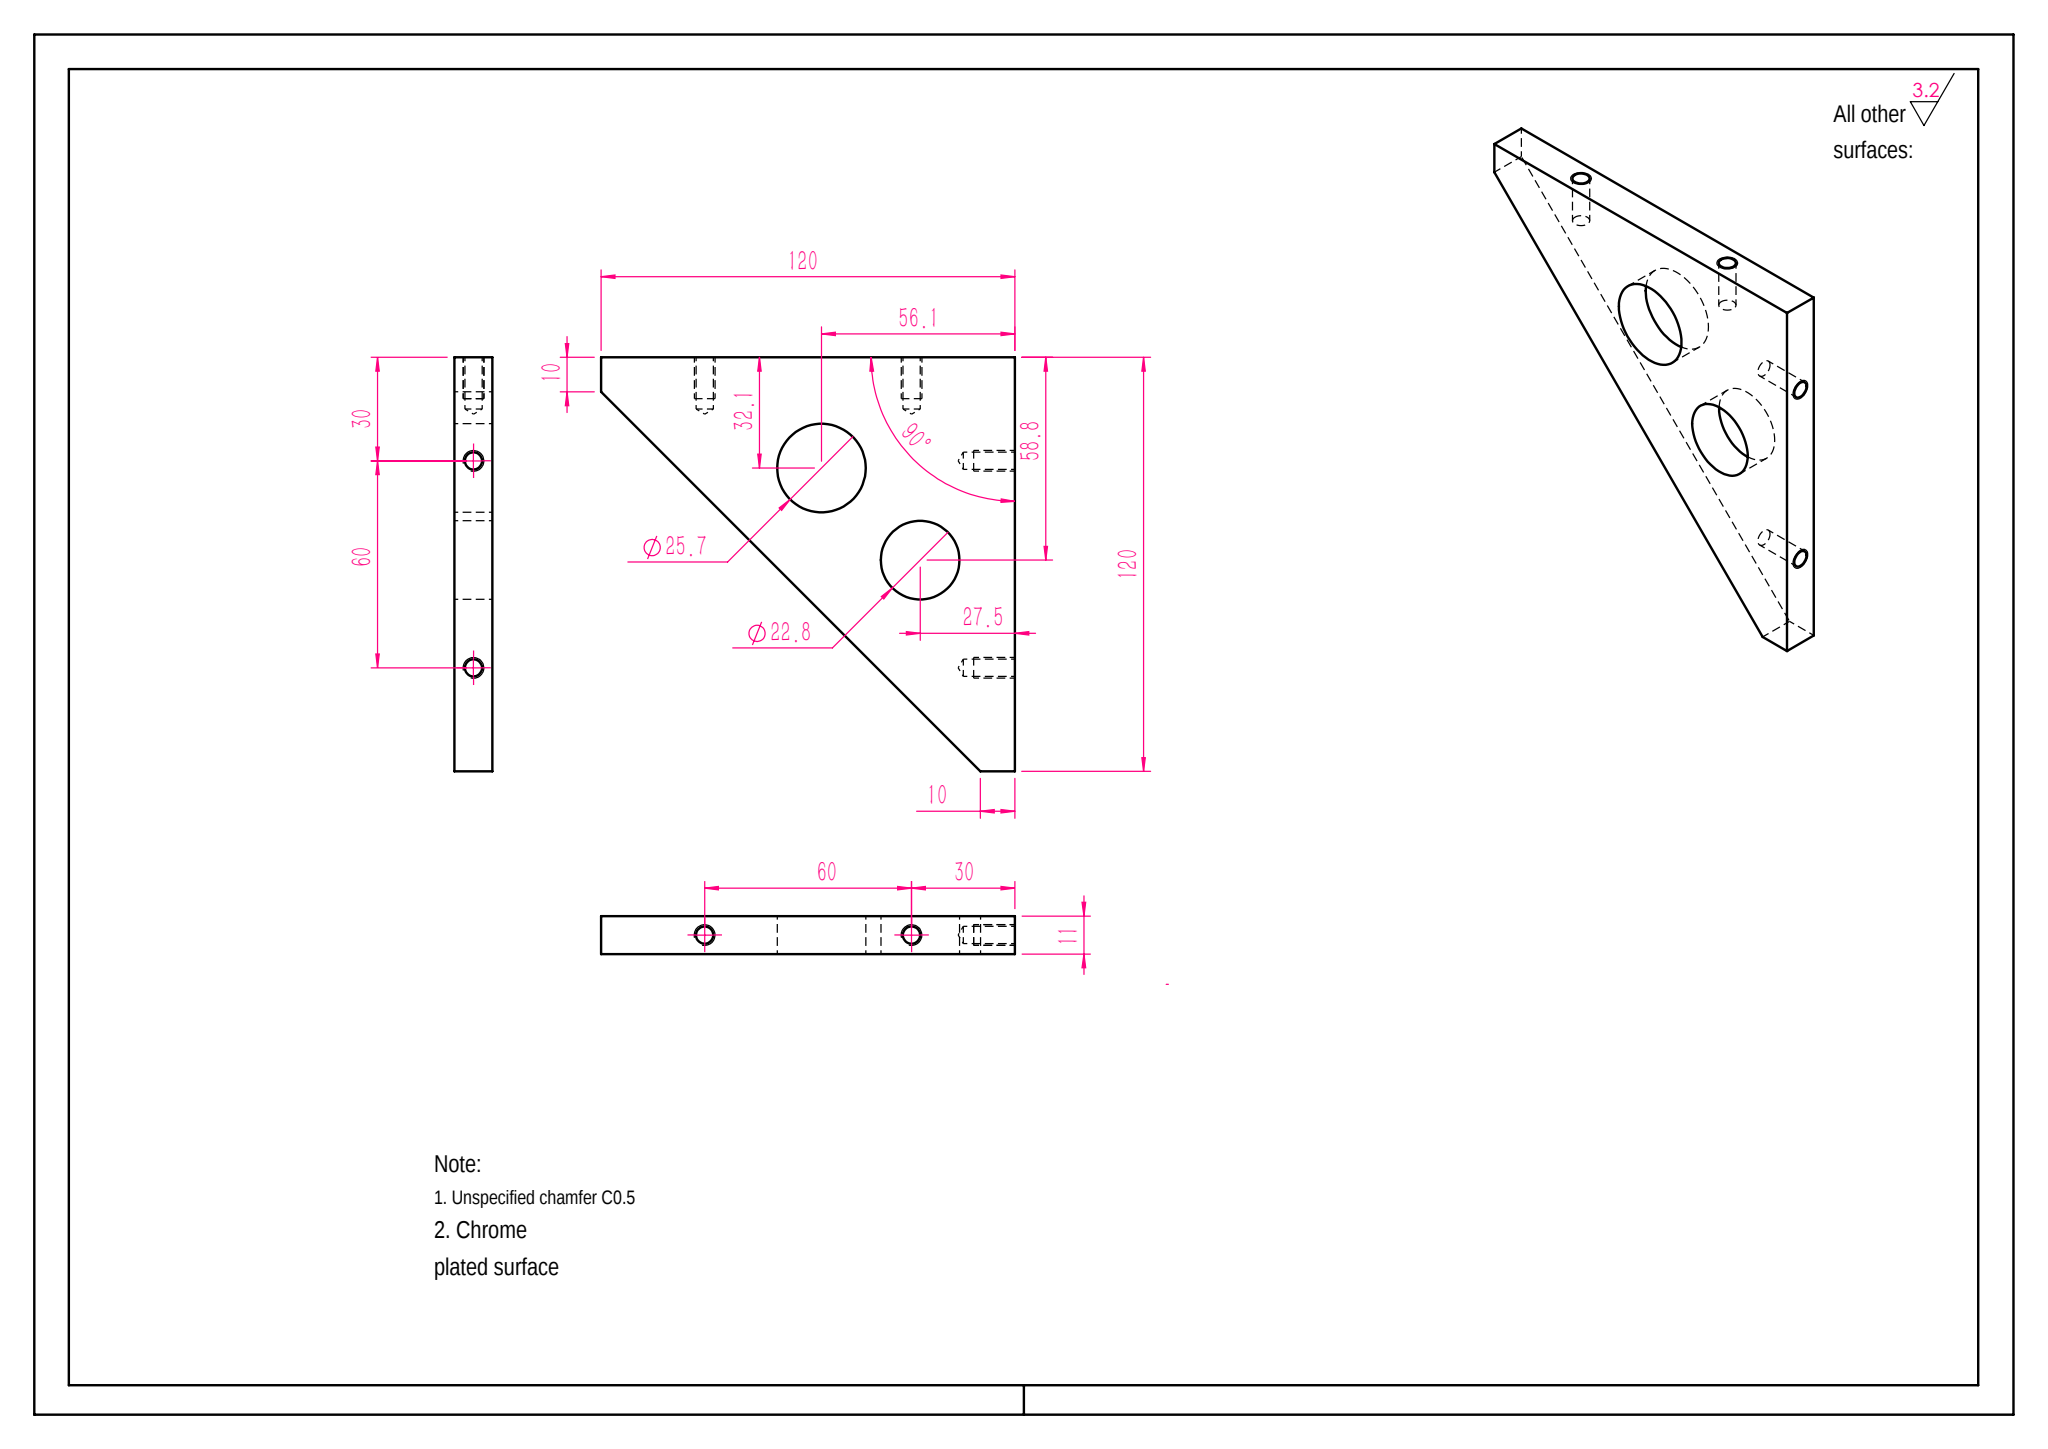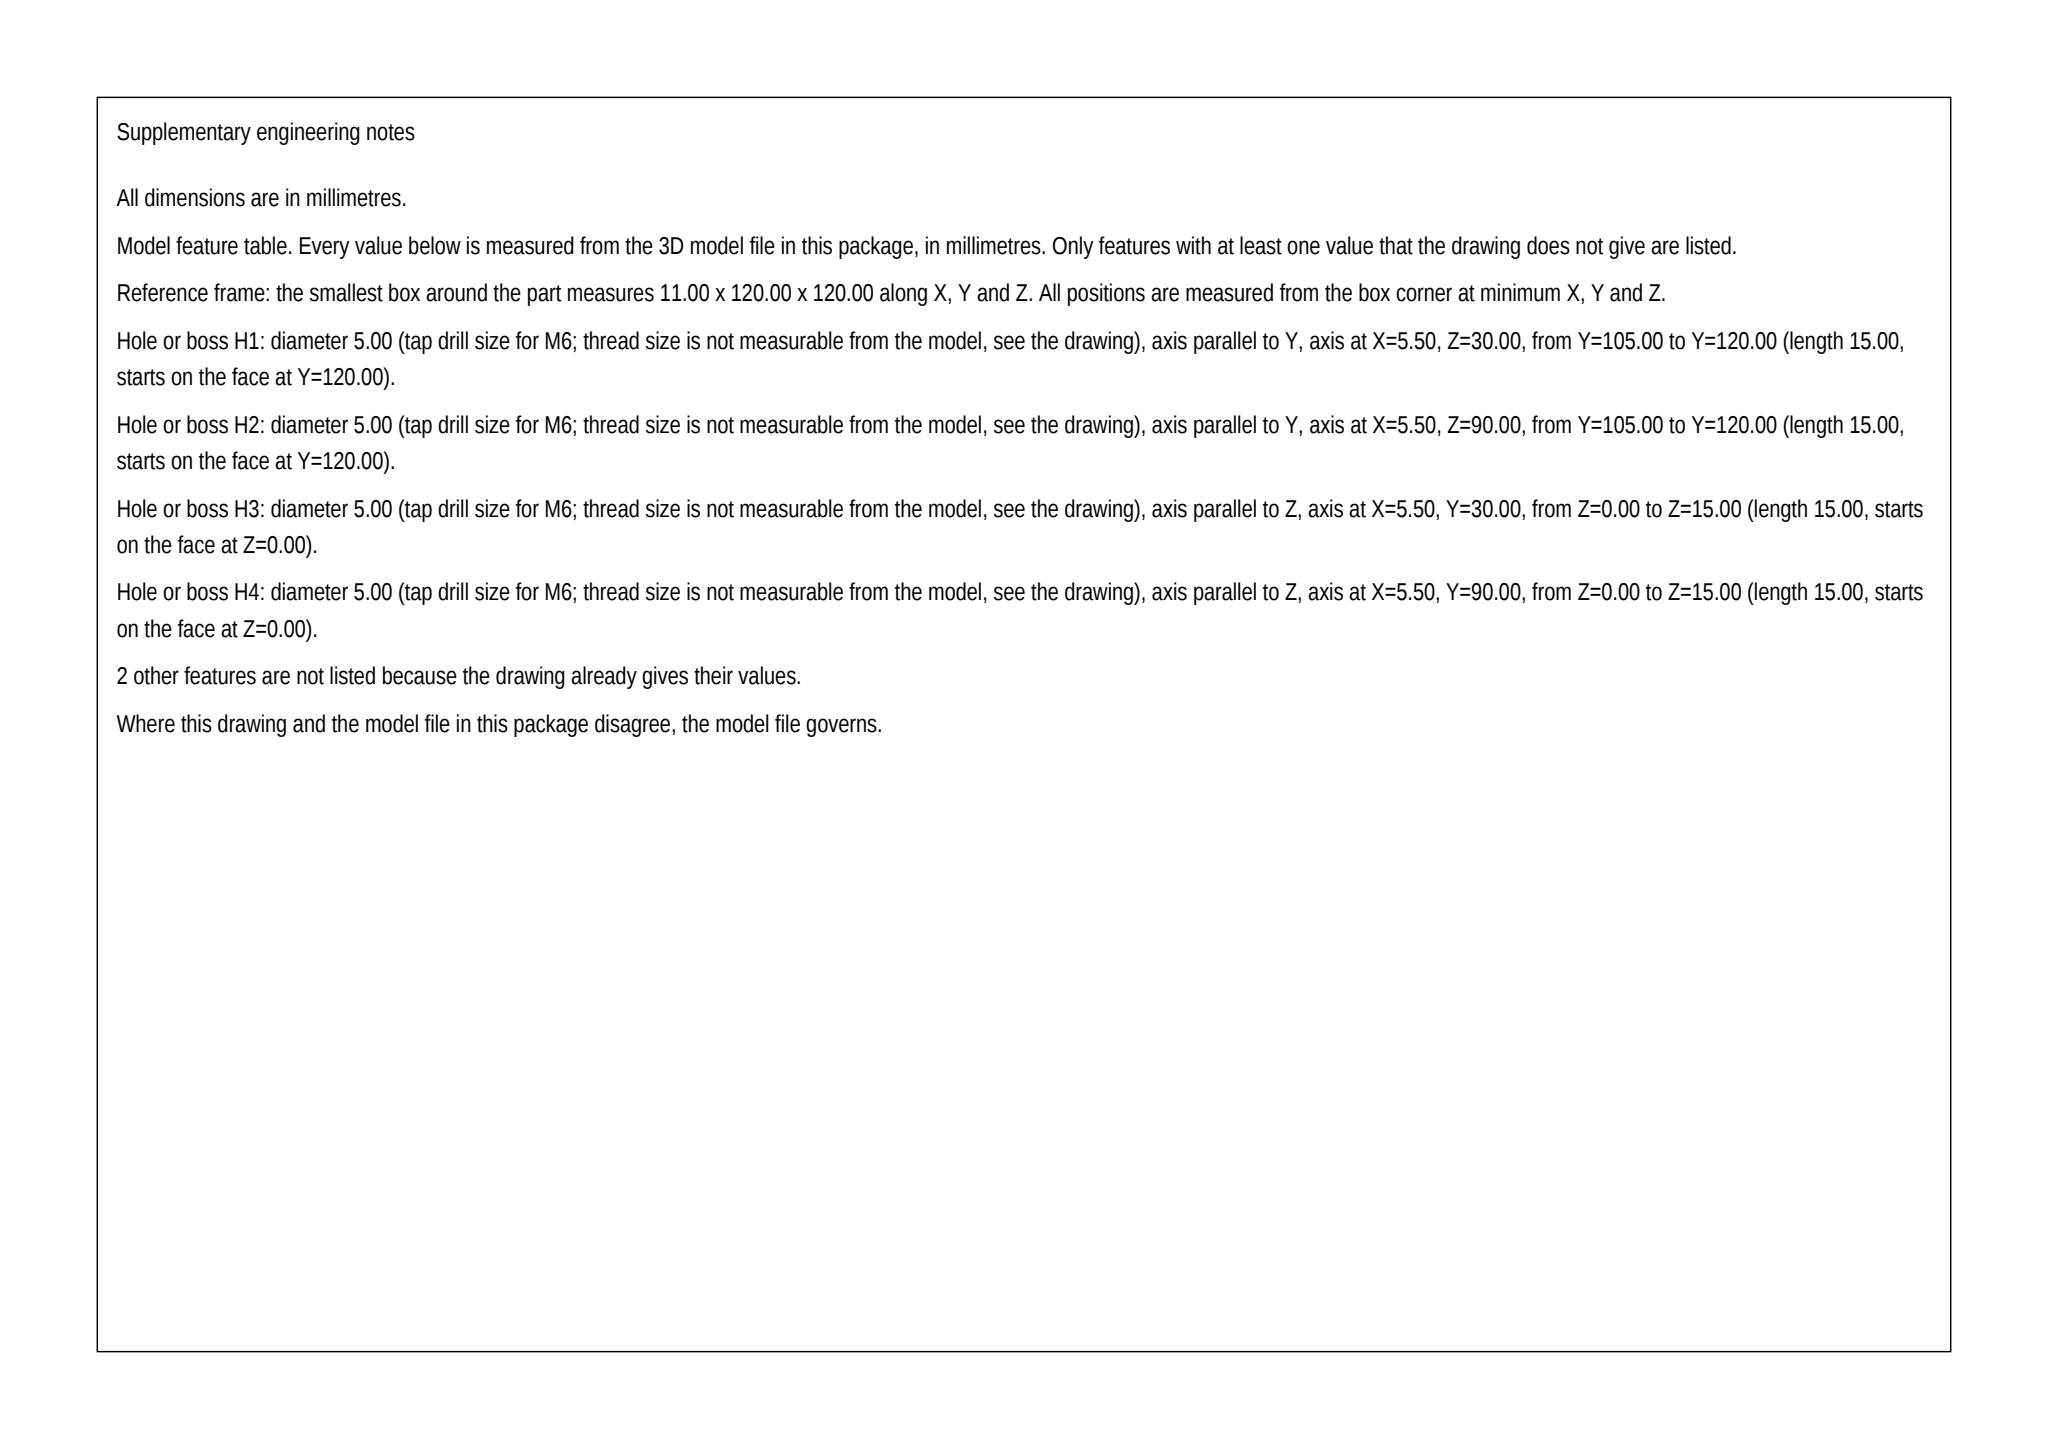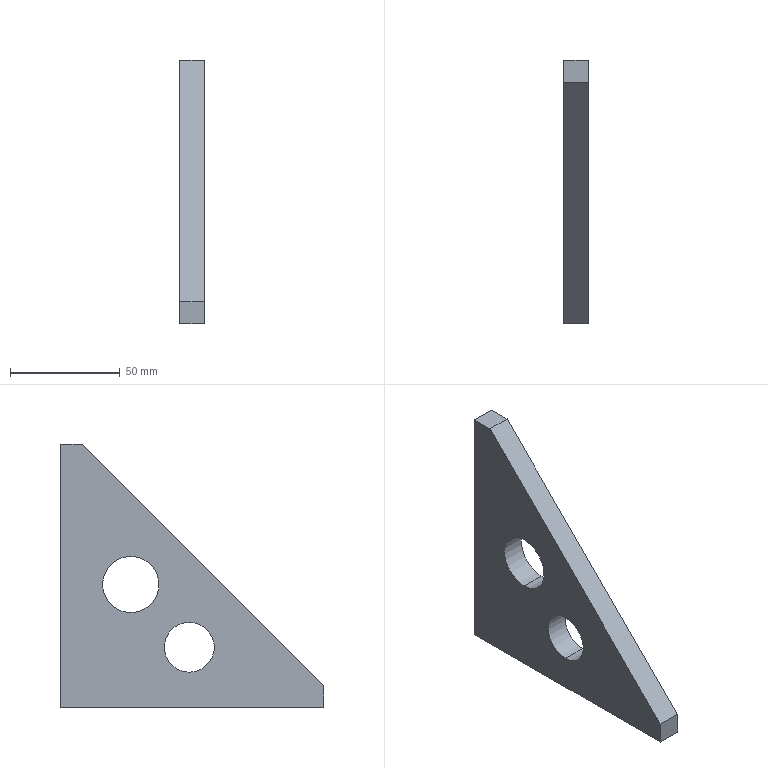Part | SolidWorks | mm | 1 solid | 27 faces | box 11 x 120 x 120 mm | volume 80448 mm3 | cylinder 12 | cone 8 | plane 7 | commonest cylinder face diameters 5 x8 22.786 x2 25.683 x2
build123d program:
from build123d import *

# Parameters (mm, degrees)
BOSS_EXTRUDE1_DEPTH   = 5.5
M6_TAPPED_HOLE1_D     = 5
M6_TAPPED_HOLE1_DEPTH = 15
M6_TAPPED_HOLE1_TIP   = 1.502
M6_TAPPED_HOLE2_D     = 5
M6_TAPPED_HOLE2_DEPTH = 15
M6_TAPPED_HOLE2_TIP   = 1.502
SKETCH6_R             = 11.393
SKETCH6_R_2           = 12.841
CUT_EXTRUDE1_DEPTH    = 80


with BuildPart() as part:
    # Sketch1 → Boss-Extrude1 (new, symmetric)
    with BuildSketch(Plane(origin=(0, 0, 0), x_dir=(0, 0, -1), z_dir=(1, 0, 0))):
        Polygon((0, 0), (0, 10), (120, 10), (120, -110), (110, -110), align=None)
    extrude(amount=BOSS_EXTRUDE1_DEPTH, both=True)

    # M6 Tapped Hole1
    with Locations(Plane(origin=(0, 0, -120), x_dir=(-1, 0, 0), z_dir=(0, 0, -1))):
        with Locations((0, -20), (0, -80)):
            Hole(M6_TAPPED_HOLE1_D / 2, depth=M6_TAPPED_HOLE1_DEPTH)
            with Locations((0, 0, -(M6_TAPPED_HOLE1_DEPTH + M6_TAPPED_HOLE1_TIP / 2))):  # 118° drill point
                Cone(0, M6_TAPPED_HOLE1_D / 2, M6_TAPPED_HOLE1_TIP, mode=Mode.SUBTRACT)

    # M6 Tapped Hole2
    with Locations(Plane(origin=(0, 10, 0), x_dir=(1, 0, 0), z_dir=(0, 1, 0))):
        with Locations((0, 90), (0, 30)):
            Hole(M6_TAPPED_HOLE2_D / 2, depth=M6_TAPPED_HOLE2_DEPTH)
            with Locations((0, 0, -(M6_TAPPED_HOLE2_DEPTH + M6_TAPPED_HOLE2_TIP / 2))):  # 118° drill point
                Cone(0, M6_TAPPED_HOLE2_D / 2, M6_TAPPED_HOLE2_TIP, mode=Mode.SUBTRACT)

    # Sketch6 → Cut-Extrude1 (cut)
    with BuildSketch(Plane.ZY.offset(5.5)):
        with Locations((-92.514, -48.763)):
            Circle(SKETCH6_R)
        with Locations((-63.888, -22.08)):
            Circle(SKETCH6_R_2)
    extrude(amount=-CUT_EXTRUDE1_DEPTH, mode=Mode.SUBTRACT)


solid = part.part
STEP:
#1=CARTESIAN_POINT('',(5.5,-48.763,-103.907));
#2=VERTEX_POINT('',#1);
#3=CARTESIAN_POINT('',(5.5,-48.763,-81.121));
#4=VERTEX_POINT('',#3);
#5=CARTESIAN_POINT('',(5.5,-48.763,-92.514));
#6=DIRECTION('',(-1.,0.,0.));
#7=DIRECTION('',(0.,0.,1.));
#8=AXIS2_PLACEMENT_3D('',#5,#6,#7);
#9=CIRCLE('',#8,11.393);
#10=EDGE_CURVE('',#2,#4,#9,.T.);
#11=ORIENTED_EDGE('',*,*,#10,.F.);
#12=CARTESIAN_POINT('',(-5.5,-48.763,-103.907));
#13=VERTEX_POINT('',#12);
#14=CARTESIAN_POINT('',(74.5,-48.763,-103.907));
#15=DIRECTION('',(-1.,0.,0.));
#16=VECTOR('',#15,1000.);
#17=LINE('',#14,#16);
#18=EDGE_CURVE('',#2,#13,#17,.T.);
#19=ORIENTED_EDGE('',*,*,#18,.T.);
#20=CARTESIAN_POINT('',(-5.5,-48.763,-81.121));
#21=VERTEX_POINT('',#20);
#22=CARTESIAN_POINT('',(-5.5,-48.763,-92.514));
#23=DIRECTION('',(-1.,0.,0.));
#24=DIRECTION('',(0.,0.,1.));
#25=AXIS2_PLACEMENT_3D('',#22,#23,#24);
#26=CIRCLE('',#25,11.393);
#27=EDGE_CURVE('',#13,#21,#26,.T.);
#28=ORIENTED_EDGE('',*,*,#27,.T.);
#29=CARTESIAN_POINT('',(74.5,-48.763,-81.121));
#30=DIRECTION('',(-1.,0.,0.));
#31=VECTOR('',#30,1000.);
#32=LINE('',#29,#31);
#33=EDGE_CURVE('',#4,#21,#32,.T.);
#34=ORIENTED_EDGE('',*,*,#33,.F.);
#35=EDGE_LOOP('',(#11,#19,#28,#34));
#36=FACE_OUTER_BOUND('',#35,.T.);
#37=CARTESIAN_POINT('',(74.5,-48.763,-92.514));
#38=DIRECTION('',(-1.,0.,0.));
#39=DIRECTION('',(0.,0.,1.));
#40=AXIS2_PLACEMENT_3D('',#37,#38,#39);
#41=CYLINDRICAL_SURFACE('',#40,11.393);
#42=ADVANCED_FACE('',(#36),#41,.F.);
#43=CARTESIAN_POINT('',(5.5,-22.08,-76.729));
#44=VERTEX_POINT('',#43);
#45=CARTESIAN_POINT('',(5.5,-22.08,-51.046));
#46=VERTEX_POINT('',#45);
#47=CARTESIAN_POINT('',(5.5,-22.08,-63.888));
#48=DIRECTION('',(-1.,0.,0.));
#49=DIRECTION('',(0.,0.,1.));
#50=AXIS2_PLACEMENT_3D('',#47,#48,#49);
#51=CIRCLE('',#50,12.841);
#52=EDGE_CURVE('',#44,#46,#51,.T.);
#53=ORIENTED_EDGE('',*,*,#52,.F.);
#54=CARTESIAN_POINT('',(-5.5,-22.08,-76.729));
#55=VERTEX_POINT('',#54);
#56=CARTESIAN_POINT('',(74.5,-22.08,-76.729));
#57=DIRECTION('',(-1.,0.,0.));
#58=VECTOR('',#57,1000.);
#59=LINE('',#56,#58);
#60=EDGE_CURVE('',#44,#55,#59,.T.);
#61=ORIENTED_EDGE('',*,*,#60,.T.);
#62=CARTESIAN_POINT('',(-5.5,-22.08,-51.046));
#63=VERTEX_POINT('',#62);
#64=CARTESIAN_POINT('',(-5.5,-22.08,-63.888));
#65=DIRECTION('',(-1.,0.,0.));
#66=DIRECTION('',(0.,0.,1.));
#67=AXIS2_PLACEMENT_3D('',#64,#65,#66);
#68=CIRCLE('',#67,12.841);
#69=EDGE_CURVE('',#55,#63,#68,.T.);
#70=ORIENTED_EDGE('',*,*,#69,.T.);
#71=CARTESIAN_POINT('',(74.5,-22.08,-51.046));
#72=DIRECTION('',(-1.,0.,0.));
#73=VECTOR('',#72,1000.);
#74=LINE('',#71,#73);
#75=EDGE_CURVE('',#46,#63,#74,.T.);
#76=ORIENTED_EDGE('',*,*,#75,.F.);
#77=EDGE_LOOP('',(#53,#61,#70,#76));
#78=FACE_OUTER_BOUND('',#77,.T.);
#79=CARTESIAN_POINT('',(74.5,-22.08,-63.888));
#80=DIRECTION('',(-1.,0.,0.));
#81=DIRECTION('',(0.,0.,1.));
#82=AXIS2_PLACEMENT_3D('',#79,#80,#81);
#83=CYLINDRICAL_SURFACE('',#82,12.841);
#84=ADVANCED_FACE('',(#78),#83,.F.);
#85=CARTESIAN_POINT('',(0.,-5.,-92.5));
#86=VERTEX_POINT('',#85);
#87=CARTESIAN_POINT('',(0.,-5.,-87.5));
#88=VERTEX_POINT('',#87);
#89=CARTESIAN_POINT('',(0.,-5.,-90.));
#90=DIRECTION('',(0.,1.,0.));
#91=DIRECTION('',(0.,0.,1.));
#92=AXIS2_PLACEMENT_3D('',#89,#90,#91);
#93=CIRCLE('',#92,2.5);
#94=EDGE_CURVE('',#86,#88,#93,.T.);
#95=ORIENTED_EDGE('',*,*,#94,.F.);
#96=CARTESIAN_POINT('',(0.,10.,-92.5));
#97=VERTEX_POINT('',#96);
#98=CARTESIAN_POINT('',(0.,10.,-92.5));
#99=DIRECTION('',(0.,1.,0.));
#100=VECTOR('',#99,1000.);
#101=LINE('',#98,#100);
#102=EDGE_CURVE('',#86,#97,#101,.T.);
#103=ORIENTED_EDGE('',*,*,#102,.T.);
#104=CARTESIAN_POINT('',(0.,10.,-87.5));
#105=VERTEX_POINT('',#104);
#106=CARTESIAN_POINT('',(0.,10.,-90.));
#107=DIRECTION('',(0.,1.,0.));
#108=DIRECTION('',(0.,0.,1.));
#109=AXIS2_PLACEMENT_3D('',#106,#107,#108);
#110=CIRCLE('',#109,2.5);
#111=EDGE_CURVE('',#97,#105,#110,.T.);
#112=ORIENTED_EDGE('',*,*,#111,.T.);
#113=CARTESIAN_POINT('',(0.,10.,-87.5));
#114=DIRECTION('',(0.,1.,0.));
#115=VECTOR('',#114,1000.);
#116=LINE('',#113,#115);
#117=EDGE_CURVE('',#88,#105,#116,.T.);
#118=ORIENTED_EDGE('',*,*,#117,.F.);
#119=EDGE_LOOP('',(#95,#103,#112,#118));
#120=FACE_OUTER_BOUND('',#119,.T.);
#121=CARTESIAN_POINT('',(0.,10.,-90.));
#122=DIRECTION('',(0.,1.,0.));
#123=DIRECTION('',(0.,0.,1.));
#124=AXIS2_PLACEMENT_3D('',#121,#122,#123);
#125=CYLINDRICAL_SURFACE('',#124,2.5);
#126=ADVANCED_FACE('',(#120),#125,.F.);
#127=CARTESIAN_POINT('',(-0.,-6.502,-90.));
#128=VERTEX_POINT('',#127);
#129=CARTESIAN_POINT('',(0.,-5.,-87.5));
#130=DIRECTION('',(0.,0.515,0.8572));
#131=VECTOR('',#130,1000.);
#132=LINE('',#129,#131);
#133=EDGE_CURVE('',#128,#88,#132,.T.);
#134=ORIENTED_EDGE('',*,*,#133,.F.);
#135=CARTESIAN_POINT('',(0.,-5.,-92.5));
#136=DIRECTION('',(0.,0.515,-0.8572));
#137=VECTOR('',#136,1000.);
#138=LINE('',#135,#137);
#139=EDGE_CURVE('',#128,#86,#138,.T.);
#140=ORIENTED_EDGE('',*,*,#139,.T.);
#141=ORIENTED_EDGE('',*,*,#94,.T.);
#142=EDGE_LOOP('',(#134,#140,#141));
#143=FACE_OUTER_BOUND('',#142,.T.);
#144=CARTESIAN_POINT('',(0.,-5.,-90.));
#145=DIRECTION('',(0.,1.,0.));
#146=DIRECTION('',(0.,0.,1.));
#147=AXIS2_PLACEMENT_3D('',#144,#145,#146);
#148=CONICAL_SURFACE('',#147,2.5,1.03);
#149=ADVANCED_FACE('',(#143),#148,.F.);
#150=CARTESIAN_POINT('',(0.,-5.,-32.5));
#151=VERTEX_POINT('',#150);
#152=CARTESIAN_POINT('',(0.,-5.,-27.5));
#153=VERTEX_POINT('',#152);
#154=CARTESIAN_POINT('',(0.,-5.,-30.));
#155=DIRECTION('',(0.,1.,0.));
#156=DIRECTION('',(0.,0.,1.));
#157=AXIS2_PLACEMENT_3D('',#154,#155,#156);
#158=CIRCLE('',#157,2.5);
#159=EDGE_CURVE('',#151,#153,#158,.T.);
#160=ORIENTED_EDGE('',*,*,#159,.F.);
#161=CARTESIAN_POINT('',(0.,10.,-32.5));
#162=VERTEX_POINT('',#161);
#163=CARTESIAN_POINT('',(0.,10.,-32.5));
#164=DIRECTION('',(0.,1.,0.));
#165=VECTOR('',#164,1000.);
#166=LINE('',#163,#165);
#167=EDGE_CURVE('',#151,#162,#166,.T.);
#168=ORIENTED_EDGE('',*,*,#167,.T.);
#169=CARTESIAN_POINT('',(0.,10.,-27.5));
#170=VERTEX_POINT('',#169);
#171=CARTESIAN_POINT('',(0.,10.,-30.));
#172=DIRECTION('',(0.,1.,0.));
#173=DIRECTION('',(0.,0.,1.));
#174=AXIS2_PLACEMENT_3D('',#171,#172,#173);
#175=CIRCLE('',#174,2.5);
#176=EDGE_CURVE('',#162,#170,#175,.T.);
#177=ORIENTED_EDGE('',*,*,#176,.T.);
#178=CARTESIAN_POINT('',(0.,10.,-27.5));
#179=DIRECTION('',(0.,1.,0.));
#180=VECTOR('',#179,1000.);
#181=LINE('',#178,#180);
#182=EDGE_CURVE('',#153,#170,#181,.T.);
#183=ORIENTED_EDGE('',*,*,#182,.F.);
#184=EDGE_LOOP('',(#160,#168,#177,#183));
#185=FACE_OUTER_BOUND('',#184,.T.);
#186=CARTESIAN_POINT('',(0.,10.,-30.));
#187=DIRECTION('',(0.,1.,0.));
#188=DIRECTION('',(0.,0.,1.));
#189=AXIS2_PLACEMENT_3D('',#186,#187,#188);
#190=CYLINDRICAL_SURFACE('',#189,2.5);
#191=ADVANCED_FACE('',(#185),#190,.F.);
#192=CARTESIAN_POINT('',(-0.,-6.502,-30.));
#193=VERTEX_POINT('',#192);
#194=CARTESIAN_POINT('',(0.,-5.,-27.5));
#195=DIRECTION('',(0.,0.515,0.8572));
#196=VECTOR('',#195,1000.);
#197=LINE('',#194,#196);
#198=EDGE_CURVE('',#193,#153,#197,.T.);
#199=ORIENTED_EDGE('',*,*,#198,.F.);
#200=CARTESIAN_POINT('',(0.,-5.,-32.5));
#201=DIRECTION('',(0.,0.515,-0.8572));
#202=VECTOR('',#201,1000.);
#203=LINE('',#200,#202);
#204=EDGE_CURVE('',#193,#151,#203,.T.);
#205=ORIENTED_EDGE('',*,*,#204,.T.);
#206=ORIENTED_EDGE('',*,*,#159,.T.);
#207=EDGE_LOOP('',(#199,#205,#206));
#208=FACE_OUTER_BOUND('',#207,.T.);
#209=CARTESIAN_POINT('',(0.,-5.,-30.));
#210=DIRECTION('',(0.,1.,0.));
#211=DIRECTION('',(0.,0.,1.));
#212=AXIS2_PLACEMENT_3D('',#209,#210,#211);
#213=CONICAL_SURFACE('',#212,2.5,1.03);
#214=ADVANCED_FACE('',(#208),#213,.F.);
#215=CARTESIAN_POINT('',(2.5,-20.,-105.));
#216=VERTEX_POINT('',#215);
#217=CARTESIAN_POINT('',(-2.5,-20.,-105.));
#218=VERTEX_POINT('',#217);
#219=CARTESIAN_POINT('',(0.,-20.,-105.));
#220=DIRECTION('',(0.,0.,-1.));
#221=DIRECTION('',(-1.,0.,0.));
#222=AXIS2_PLACEMENT_3D('',#219,#220,#221);
#223=CIRCLE('',#222,2.5);
#224=EDGE_CURVE('',#216,#218,#223,.T.);
#225=ORIENTED_EDGE('',*,*,#224,.F.);
#226=CARTESIAN_POINT('',(2.5,-20.,-120.));
#227=VERTEX_POINT('',#226);
#228=CARTESIAN_POINT('',(2.5,-20.,-120.));
#229=DIRECTION('',(0.,0.,-1.));
#230=VECTOR('',#229,1000.);
#231=LINE('',#228,#230);
#232=EDGE_CURVE('',#216,#227,#231,.T.);
#233=ORIENTED_EDGE('',*,*,#232,.T.);
#234=CARTESIAN_POINT('',(-2.5,-20.,-120.));
#235=VERTEX_POINT('',#234);
#236=CARTESIAN_POINT('',(0.,-20.,-120.));
#237=DIRECTION('',(0.,0.,-1.));
#238=DIRECTION('',(-1.,0.,0.));
#239=AXIS2_PLACEMENT_3D('',#236,#237,#238);
#240=CIRCLE('',#239,2.5);
#241=EDGE_CURVE('',#227,#235,#240,.T.);
#242=ORIENTED_EDGE('',*,*,#241,.T.);
#243=CARTESIAN_POINT('',(-2.5,-20.,-120.));
#244=DIRECTION('',(0.,0.,-1.));
#245=VECTOR('',#244,1000.);
#246=LINE('',#243,#245);
#247=EDGE_CURVE('',#218,#235,#246,.T.);
#248=ORIENTED_EDGE('',*,*,#247,.F.);
#249=EDGE_LOOP('',(#225,#233,#242,#248));
#250=FACE_OUTER_BOUND('',#249,.T.);
#251=CARTESIAN_POINT('',(0.,-20.,-120.));
#252=DIRECTION('',(0.,0.,-1.));
#253=DIRECTION('',(-1.,0.,0.));
#254=AXIS2_PLACEMENT_3D('',#251,#252,#253);
#255=CYLINDRICAL_SURFACE('',#254,2.5);
#256=ADVANCED_FACE('',(#250),#255,.F.);
#257=CARTESIAN_POINT('',(-0.,-20.,-103.498));
#258=VERTEX_POINT('',#257);
#259=CARTESIAN_POINT('',(-2.5,-20.,-105.));
#260=DIRECTION('',(-0.8572,0.,-0.515));
#261=VECTOR('',#260,1000.);
#262=LINE('',#259,#261);
#263=EDGE_CURVE('',#258,#218,#262,.T.);
#264=ORIENTED_EDGE('',*,*,#263,.F.);
#265=CARTESIAN_POINT('',(2.5,-20.,-105.));
#266=DIRECTION('',(0.8572,0.,-0.515));
#267=VECTOR('',#266,1000.);
#268=LINE('',#265,#267);
#269=EDGE_CURVE('',#258,#216,#268,.T.);
#270=ORIENTED_EDGE('',*,*,#269,.T.);
#271=ORIENTED_EDGE('',*,*,#224,.T.);
#272=EDGE_LOOP('',(#264,#270,#271));
#273=FACE_OUTER_BOUND('',#272,.T.);
#274=CARTESIAN_POINT('',(0.,-20.,-105.));
#275=DIRECTION('',(0.,0.,-1.));
#276=DIRECTION('',(-1.,0.,0.));
#277=AXIS2_PLACEMENT_3D('',#274,#275,#276);
#278=CONICAL_SURFACE('',#277,2.5,1.03);
#279=ADVANCED_FACE('',(#273),#278,.F.);
#280=CARTESIAN_POINT('',(2.5,-80.,-105.));
#281=VERTEX_POINT('',#280);
#282=CARTESIAN_POINT('',(-2.5,-80.,-105.));
#283=VERTEX_POINT('',#282);
#284=CARTESIAN_POINT('',(0.,-80.,-105.));
#285=DIRECTION('',(0.,0.,-1.));
#286=DIRECTION('',(-1.,0.,0.));
#287=AXIS2_PLACEMENT_3D('',#284,#285,#286);
#288=CIRCLE('',#287,2.5);
#289=EDGE_CURVE('',#281,#283,#288,.T.);
#290=ORIENTED_EDGE('',*,*,#289,.F.);
#291=CARTESIAN_POINT('',(2.5,-80.,-120.));
#292=VERTEX_POINT('',#291);
#293=CARTESIAN_POINT('',(2.5,-80.,-120.));
#294=DIRECTION('',(0.,0.,-1.));
#295=VECTOR('',#294,1000.);
#296=LINE('',#293,#295);
#297=EDGE_CURVE('',#281,#292,#296,.T.);
#298=ORIENTED_EDGE('',*,*,#297,.T.);
#299=CARTESIAN_POINT('',(-2.5,-80.,-120.));
#300=VERTEX_POINT('',#299);
#301=CARTESIAN_POINT('',(0.,-80.,-120.));
#302=DIRECTION('',(0.,0.,-1.));
#303=DIRECTION('',(-1.,0.,0.));
#304=AXIS2_PLACEMENT_3D('',#301,#302,#303);
#305=CIRCLE('',#304,2.5);
#306=EDGE_CURVE('',#292,#300,#305,.T.);
#307=ORIENTED_EDGE('',*,*,#306,.T.);
#308=CARTESIAN_POINT('',(-2.5,-80.,-120.));
#309=DIRECTION('',(0.,0.,-1.));
#310=VECTOR('',#309,1000.);
#311=LINE('',#308,#310);
#312=EDGE_CURVE('',#283,#300,#311,.T.);
#313=ORIENTED_EDGE('',*,*,#312,.F.);
#314=EDGE_LOOP('',(#290,#298,#307,#313));
#315=FACE_OUTER_BOUND('',#314,.T.);
#316=CARTESIAN_POINT('',(0.,-80.,-120.));
#317=DIRECTION('',(0.,0.,-1.));
#318=DIRECTION('',(-1.,0.,0.));
#319=AXIS2_PLACEMENT_3D('',#316,#317,#318);
#320=CYLINDRICAL_SURFACE('',#319,2.5);
#321=ADVANCED_FACE('',(#315),#320,.F.);
#322=CARTESIAN_POINT('',(-0.,-80.,-103.498));
#323=VERTEX_POINT('',#322);
#324=CARTESIAN_POINT('',(-2.5,-80.,-105.));
#325=DIRECTION('',(-0.8572,0.,-0.515));
#326=VECTOR('',#325,1000.);
#327=LINE('',#324,#326);
#328=EDGE_CURVE('',#323,#283,#327,.T.);
#329=ORIENTED_EDGE('',*,*,#328,.F.);
#330=CARTESIAN_POINT('',(2.5,-80.,-105.));
#331=DIRECTION('',(0.8572,0.,-0.515));
#332=VECTOR('',#331,1000.);
#333=LINE('',#330,#332);
#334=EDGE_CURVE('',#323,#281,#333,.T.);
#335=ORIENTED_EDGE('',*,*,#334,.T.);
#336=ORIENTED_EDGE('',*,*,#289,.T.);
#337=EDGE_LOOP('',(#329,#335,#336));
#338=FACE_OUTER_BOUND('',#337,.T.);
#339=CARTESIAN_POINT('',(0.,-80.,-105.));
#340=DIRECTION('',(0.,0.,-1.));
#341=DIRECTION('',(-1.,0.,0.));
#342=AXIS2_PLACEMENT_3D('',#339,#340,#341);
#343=CONICAL_SURFACE('',#342,2.5,1.03);
#344=ADVANCED_FACE('',(#338),#343,.F.);
#345=CARTESIAN_POINT('',(-5.5,0.,0.));
#346=VERTEX_POINT('',#345);
#347=CARTESIAN_POINT('',(-5.5,-110.,-110.));
#348=VERTEX_POINT('',#347);
#349=CARTESIAN_POINT('',(-5.5,-110.,-110.));
#350=DIRECTION('',(0.,-0.7071,-0.7071));
#351=VECTOR('',#350,1000.);
#352=LINE('',#349,#351);
#353=EDGE_CURVE('',#346,#348,#352,.T.);
#354=ORIENTED_EDGE('',*,*,#353,.T.);
#355=CARTESIAN_POINT('',(5.5,-110.,-110.));
#356=VERTEX_POINT('',#355);
#357=CARTESIAN_POINT('',(5.5,-110.,-110.));
#358=DIRECTION('',(-1.,0.,0.));
#359=VECTOR('',#358,1000.);
#360=LINE('',#357,#359);
#361=EDGE_CURVE('',#356,#348,#360,.T.);
#362=ORIENTED_EDGE('',*,*,#361,.F.);
#363=CARTESIAN_POINT('',(5.5,0.,0.));
#364=VERTEX_POINT('',#363);
#365=CARTESIAN_POINT('',(5.5,-110.,-110.));
#366=DIRECTION('',(0.,-0.7071,-0.7071));
#367=VECTOR('',#366,1000.);
#368=LINE('',#365,#367);
#369=EDGE_CURVE('',#364,#356,#368,.T.);
#370=ORIENTED_EDGE('',*,*,#369,.F.);
#371=CARTESIAN_POINT('',(5.5,0.,0.));
#372=DIRECTION('',(-1.,0.,0.));
#373=VECTOR('',#372,1000.);
#374=LINE('',#371,#373);
#375=EDGE_CURVE('',#364,#346,#374,.T.);
#376=ORIENTED_EDGE('',*,*,#375,.T.);
#377=EDGE_LOOP('',(#354,#362,#370,#376));
#378=FACE_OUTER_BOUND('',#377,.T.);
#379=CARTESIAN_POINT('',(5.5,-110.,-110.));
#380=DIRECTION('',(0.,0.7071,-0.7071));
#381=DIRECTION('',(0.,0.7071,0.7071));
#382=AXIS2_PLACEMENT_3D('',#379,#380,#381);
#383=PLANE('',#382);
#384=ADVANCED_FACE('',(#378),#383,.F.);
#385=CARTESIAN_POINT('',(-5.5,-110.,-120.));
#386=VERTEX_POINT('',#385);
#387=CARTESIAN_POINT('',(-5.5,-110.,-120.));
#388=DIRECTION('',(0.,-0.,-1.));
#389=VECTOR('',#388,1000.);
#390=LINE('',#387,#389);
#391=EDGE_CURVE('',#348,#386,#390,.T.);
#392=ORIENTED_EDGE('',*,*,#391,.T.);
#393=CARTESIAN_POINT('',(5.5,-110.,-120.));
#394=VERTEX_POINT('',#393);
#395=CARTESIAN_POINT('',(5.5,-110.,-120.));
#396=DIRECTION('',(-1.,0.,0.));
#397=VECTOR('',#396,1000.);
#398=LINE('',#395,#397);
#399=EDGE_CURVE('',#394,#386,#398,.T.);
#400=ORIENTED_EDGE('',*,*,#399,.F.);
#401=CARTESIAN_POINT('',(5.5,-110.,-120.));
#402=DIRECTION('',(0.,-0.,-1.));
#403=VECTOR('',#402,1000.);
#404=LINE('',#401,#403);
#405=EDGE_CURVE('',#356,#394,#404,.T.);
#406=ORIENTED_EDGE('',*,*,#405,.F.);
#407=ORIENTED_EDGE('',*,*,#361,.T.);
#408=EDGE_LOOP('',(#392,#400,#406,#407));
#409=FACE_OUTER_BOUND('',#408,.T.);
#410=CARTESIAN_POINT('',(5.5,-110.,-120.));
#411=DIRECTION('',(0.,1.,-0.));
#412=DIRECTION('',(0.,0.,1.));
#413=AXIS2_PLACEMENT_3D('',#410,#411,#412);
#414=PLANE('',#413);
#415=ADVANCED_FACE('',(#409),#414,.F.);
#416=CARTESIAN_POINT('',(0.,-20.,-120.));
#417=DIRECTION('',(0.,0.,-1.));
#418=DIRECTION('',(-1.,0.,0.));
#419=AXIS2_PLACEMENT_3D('',#416,#417,#418);
#420=CIRCLE('',#419,2.5);
#421=EDGE_CURVE('',#235,#227,#420,.T.);
#422=ORIENTED_EDGE('',*,*,#421,.F.);
#423=ORIENTED_EDGE('',*,*,#241,.F.);
#424=EDGE_LOOP('',(#422,#423));
#425=FACE_BOUND('',#424,.T.);
#426=CARTESIAN_POINT('',(0.,-80.,-120.));
#427=DIRECTION('',(0.,0.,-1.));
#428=DIRECTION('',(-1.,0.,0.));
#429=AXIS2_PLACEMENT_3D('',#426,#427,#428);
#430=CIRCLE('',#429,2.5);
#431=EDGE_CURVE('',#300,#292,#430,.T.);
#432=ORIENTED_EDGE('',*,*,#431,.F.);
#433=ORIENTED_EDGE('',*,*,#306,.F.);
#434=EDGE_LOOP('',(#432,#433));
#435=FACE_BOUND('',#434,.T.);
#436=CARTESIAN_POINT('',(-5.5,10.,-120.));
#437=VERTEX_POINT('',#436);
#438=CARTESIAN_POINT('',(-5.5,10.,-120.));
#439=DIRECTION('',(0.,1.,0.));
#440=VECTOR('',#439,1000.);
#441=LINE('',#438,#440);
#442=EDGE_CURVE('',#386,#437,#441,.T.);
#443=ORIENTED_EDGE('',*,*,#442,.T.);
#444=CARTESIAN_POINT('',(5.5,10.,-120.));
#445=VERTEX_POINT('',#444);
#446=CARTESIAN_POINT('',(5.5,10.,-120.));
#447=DIRECTION('',(-1.,0.,0.));
#448=VECTOR('',#447,1000.);
#449=LINE('',#446,#448);
#450=EDGE_CURVE('',#445,#437,#449,.T.);
#451=ORIENTED_EDGE('',*,*,#450,.F.);
#452=CARTESIAN_POINT('',(5.5,10.,-120.));
#453=DIRECTION('',(0.,1.,0.));
#454=VECTOR('',#453,1000.);
#455=LINE('',#452,#454);
#456=EDGE_CURVE('',#394,#445,#455,.T.);
#457=ORIENTED_EDGE('',*,*,#456,.F.);
#458=ORIENTED_EDGE('',*,*,#399,.T.);
#459=EDGE_LOOP('',(#443,#451,#457,#458));
#460=FACE_OUTER_BOUND('',#459,.T.);
#461=CARTESIAN_POINT('',(5.5,10.,-120.));
#462=DIRECTION('',(0.,0.,1.));
#463=DIRECTION('',(1.,0.,0.));
#464=AXIS2_PLACEMENT_3D('',#461,#462,#463);
#465=PLANE('',#464);
#466=ADVANCED_FACE('',(#425,#435,#460),#465,.F.);
#467=CARTESIAN_POINT('',(0.,10.,-90.));
#468=DIRECTION('',(0.,1.,0.));
#469=DIRECTION('',(0.,0.,1.));
#470=AXIS2_PLACEMENT_3D('',#467,#468,#469);
#471=CIRCLE('',#470,2.5);
#472=EDGE_CURVE('',#105,#97,#471,.T.);
#473=ORIENTED_EDGE('',*,*,#472,.F.);
#474=ORIENTED_EDGE('',*,*,#111,.F.);
#475=EDGE_LOOP('',(#473,#474));
#476=FACE_BOUND('',#475,.T.);
#477=CARTESIAN_POINT('',(0.,10.,-30.));
#478=DIRECTION('',(0.,1.,0.));
#479=DIRECTION('',(0.,0.,1.));
#480=AXIS2_PLACEMENT_3D('',#477,#478,#479);
#481=CIRCLE('',#480,2.5);
#482=EDGE_CURVE('',#170,#162,#481,.T.);
#483=ORIENTED_EDGE('',*,*,#482,.F.);
#484=ORIENTED_EDGE('',*,*,#176,.F.);
#485=EDGE_LOOP('',(#483,#484));
#486=FACE_BOUND('',#485,.T.);
#487=CARTESIAN_POINT('',(-5.5,10.,0.));
#488=VERTEX_POINT('',#487);
#489=CARTESIAN_POINT('',(-5.5,10.,0.));
#490=DIRECTION('',(0.,0.,1.));
#491=VECTOR('',#490,1000.);
#492=LINE('',#489,#491);
#493=EDGE_CURVE('',#437,#488,#492,.T.);
#494=ORIENTED_EDGE('',*,*,#493,.T.);
#495=CARTESIAN_POINT('',(5.5,10.,0.));
#496=VERTEX_POINT('',#495);
#497=CARTESIAN_POINT('',(5.5,10.,0.));
#498=DIRECTION('',(-1.,0.,0.));
#499=VECTOR('',#498,1000.);
#500=LINE('',#497,#499);
#501=EDGE_CURVE('',#496,#488,#500,.T.);
#502=ORIENTED_EDGE('',*,*,#501,.F.);
#503=CARTESIAN_POINT('',(5.5,10.,0.));
#504=DIRECTION('',(0.,0.,1.));
#505=VECTOR('',#504,1000.);
#506=LINE('',#503,#505);
#507=EDGE_CURVE('',#445,#496,#506,.T.);
#508=ORIENTED_EDGE('',*,*,#507,.F.);
#509=ORIENTED_EDGE('',*,*,#450,.T.);
#510=EDGE_LOOP('',(#494,#502,#508,#509));
#511=FACE_OUTER_BOUND('',#510,.T.);
#512=CARTESIAN_POINT('',(5.5,10.,0.));
#513=DIRECTION('',(0.,-1.,0.));
#514=DIRECTION('',(0.,0.,-1.));
#515=AXIS2_PLACEMENT_3D('',#512,#513,#514);
#516=PLANE('',#515);
#517=ADVANCED_FACE('',(#476,#486,#511),#516,.F.);
#518=CARTESIAN_POINT('',(-5.5,0.,0.));
#519=DIRECTION('',(0.,-1.,0.));
#520=VECTOR('',#519,1000.);
#521=LINE('',#518,#520);
#522=EDGE_CURVE('',#488,#346,#521,.T.);
#523=ORIENTED_EDGE('',*,*,#522,.T.);
#524=ORIENTED_EDGE('',*,*,#375,.F.);
#525=CARTESIAN_POINT('',(5.5,0.,0.));
#526=DIRECTION('',(0.,-1.,0.));
#527=VECTOR('',#526,1000.);
#528=LINE('',#525,#527);
#529=EDGE_CURVE('',#496,#364,#528,.T.);
#530=ORIENTED_EDGE('',*,*,#529,.F.);
#531=ORIENTED_EDGE('',*,*,#501,.T.);
#532=EDGE_LOOP('',(#523,#524,#530,#531));
#533=FACE_OUTER_BOUND('',#532,.T.);
#534=CARTESIAN_POINT('',(5.5,0.,0.));
#535=DIRECTION('',(0.,0.,-1.));
#536=DIRECTION('',(-1.,0.,0.));
#537=AXIS2_PLACEMENT_3D('',#534,#535,#536);
#538=PLANE('',#537);
#539=ADVANCED_FACE('',(#533),#538,.F.);
#540=CARTESIAN_POINT('',(5.5,-48.763,-92.514));
#541=DIRECTION('',(-1.,0.,0.));
#542=DIRECTION('',(0.,0.,1.));
#543=AXIS2_PLACEMENT_3D('',#540,#541,#542);
#544=CIRCLE('',#543,11.393);
#545=EDGE_CURVE('',#4,#2,#544,.T.);
#546=ORIENTED_EDGE('',*,*,#545,.T.);
#547=ORIENTED_EDGE('',*,*,#10,.T.);
#548=EDGE_LOOP('',(#546,#547));
#549=FACE_BOUND('',#548,.T.);
#550=CARTESIAN_POINT('',(5.5,-22.08,-63.888));
#551=DIRECTION('',(-1.,0.,0.));
#552=DIRECTION('',(0.,0.,1.));
#553=AXIS2_PLACEMENT_3D('',#550,#551,#552);
#554=CIRCLE('',#553,12.841);
#555=EDGE_CURVE('',#46,#44,#554,.T.);
#556=ORIENTED_EDGE('',*,*,#555,.T.);
#557=ORIENTED_EDGE('',*,*,#52,.T.);
#558=EDGE_LOOP('',(#556,#557));
#559=FACE_BOUND('',#558,.T.);
#560=ORIENTED_EDGE('',*,*,#369,.T.);
#561=ORIENTED_EDGE('',*,*,#405,.T.);
#562=ORIENTED_EDGE('',*,*,#456,.T.);
#563=ORIENTED_EDGE('',*,*,#507,.T.);
#564=ORIENTED_EDGE('',*,*,#529,.T.);
#565=EDGE_LOOP('',(#560,#561,#562,#563,#564));
#566=FACE_OUTER_BOUND('',#565,.T.);
#567=CARTESIAN_POINT('',(5.5,0.,0.));
#568=DIRECTION('',(-1.,0.,0.));
#569=DIRECTION('',(0.,0.,1.));
#570=AXIS2_PLACEMENT_3D('',#567,#568,#569);
#571=PLANE('',#570);
#572=ADVANCED_FACE('',(#549,#559,#566),#571,.F.);
#573=CARTESIAN_POINT('',(-5.5,-48.763,-92.514));
#574=DIRECTION('',(-1.,0.,0.));
#575=DIRECTION('',(0.,0.,1.));
#576=AXIS2_PLACEMENT_3D('',#573,#574,#575);
#577=CIRCLE('',#576,11.393);
#578=EDGE_CURVE('',#21,#13,#577,.T.);
#579=ORIENTED_EDGE('',*,*,#578,.F.);
#580=ORIENTED_EDGE('',*,*,#27,.F.);
#581=EDGE_LOOP('',(#579,#580));
#582=FACE_BOUND('',#581,.T.);
#583=CARTESIAN_POINT('',(-5.5,-22.08,-63.888));
#584=DIRECTION('',(-1.,0.,0.));
#585=DIRECTION('',(0.,0.,1.));
#586=AXIS2_PLACEMENT_3D('',#583,#584,#585);
#587=CIRCLE('',#586,12.841);
#588=EDGE_CURVE('',#63,#55,#587,.T.);
#589=ORIENTED_EDGE('',*,*,#588,.F.);
#590=ORIENTED_EDGE('',*,*,#69,.F.);
#591=EDGE_LOOP('',(#589,#590));
#592=FACE_BOUND('',#591,.T.);
#593=ORIENTED_EDGE('',*,*,#353,.F.);
#594=ORIENTED_EDGE('',*,*,#522,.F.);
#595=ORIENTED_EDGE('',*,*,#493,.F.);
#596=ORIENTED_EDGE('',*,*,#442,.F.);
#597=ORIENTED_EDGE('',*,*,#391,.F.);
#598=EDGE_LOOP('',(#593,#594,#595,#596,#597));
#599=FACE_OUTER_BOUND('',#598,.T.);
#600=CARTESIAN_POINT('',(-5.5,0.,0.));
#601=DIRECTION('',(-1.,0.,0.));
#602=DIRECTION('',(0.,0.,1.));
#603=AXIS2_PLACEMENT_3D('',#600,#601,#602);
#604=PLANE('',#603);
#605=ADVANCED_FACE('',(#582,#592,#599),#604,.T.);
#606=ORIENTED_EDGE('',*,*,#334,.F.);
#607=ORIENTED_EDGE('',*,*,#328,.T.);
#608=CARTESIAN_POINT('',(0.,-80.,-105.));
#609=DIRECTION('',(0.,0.,-1.));
#610=DIRECTION('',(-1.,0.,0.));
#611=AXIS2_PLACEMENT_3D('',#608,#609,#610);
#612=CIRCLE('',#611,2.5);
#613=EDGE_CURVE('',#283,#281,#612,.T.);
#614=ORIENTED_EDGE('',*,*,#613,.T.);
#615=EDGE_LOOP('',(#606,#607,#614));
#616=FACE_OUTER_BOUND('',#615,.T.);
#617=CARTESIAN_POINT('',(0.,-80.,-105.));
#618=DIRECTION('',(0.,0.,-1.));
#619=DIRECTION('',(-1.,0.,0.));
#620=AXIS2_PLACEMENT_3D('',#617,#618,#619);
#621=CONICAL_SURFACE('',#620,2.5,1.03);
#622=ADVANCED_FACE('',(#616),#621,.F.);
#623=ORIENTED_EDGE('',*,*,#297,.F.);
#624=ORIENTED_EDGE('',*,*,#613,.F.);
#625=ORIENTED_EDGE('',*,*,#312,.T.);
#626=ORIENTED_EDGE('',*,*,#431,.T.);
#627=EDGE_LOOP('',(#623,#624,#625,#626));
#628=FACE_OUTER_BOUND('',#627,.T.);
#629=CARTESIAN_POINT('',(0.,-80.,-120.));
#630=DIRECTION('',(0.,0.,-1.));
#631=DIRECTION('',(-1.,0.,0.));
#632=AXIS2_PLACEMENT_3D('',#629,#630,#631);
#633=CYLINDRICAL_SURFACE('',#632,2.5);
#634=ADVANCED_FACE('',(#628),#633,.F.);
#635=ORIENTED_EDGE('',*,*,#269,.F.);
#636=ORIENTED_EDGE('',*,*,#263,.T.);
#637=CARTESIAN_POINT('',(0.,-20.,-105.));
#638=DIRECTION('',(0.,0.,-1.));
#639=DIRECTION('',(-1.,0.,0.));
#640=AXIS2_PLACEMENT_3D('',#637,#638,#639);
#641=CIRCLE('',#640,2.5);
#642=EDGE_CURVE('',#218,#216,#641,.T.);
#643=ORIENTED_EDGE('',*,*,#642,.T.);
#644=EDGE_LOOP('',(#635,#636,#643));
#645=FACE_OUTER_BOUND('',#644,.T.);
#646=CARTESIAN_POINT('',(0.,-20.,-105.));
#647=DIRECTION('',(0.,0.,-1.));
#648=DIRECTION('',(-1.,0.,0.));
#649=AXIS2_PLACEMENT_3D('',#646,#647,#648);
#650=CONICAL_SURFACE('',#649,2.5,1.03);
#651=ADVANCED_FACE('',(#645),#650,.F.);
#652=ORIENTED_EDGE('',*,*,#232,.F.);
#653=ORIENTED_EDGE('',*,*,#642,.F.);
#654=ORIENTED_EDGE('',*,*,#247,.T.);
#655=ORIENTED_EDGE('',*,*,#421,.T.);
#656=EDGE_LOOP('',(#652,#653,#654,#655));
#657=FACE_OUTER_BOUND('',#656,.T.);
#658=CARTESIAN_POINT('',(0.,-20.,-120.));
#659=DIRECTION('',(0.,0.,-1.));
#660=DIRECTION('',(-1.,0.,0.));
#661=AXIS2_PLACEMENT_3D('',#658,#659,#660);
#662=CYLINDRICAL_SURFACE('',#661,2.5);
#663=ADVANCED_FACE('',(#657),#662,.F.);
#664=ORIENTED_EDGE('',*,*,#204,.F.);
#665=ORIENTED_EDGE('',*,*,#198,.T.);
#666=CARTESIAN_POINT('',(0.,-5.,-30.));
#667=DIRECTION('',(0.,1.,0.));
#668=DIRECTION('',(0.,0.,1.));
#669=AXIS2_PLACEMENT_3D('',#666,#667,#668);
#670=CIRCLE('',#669,2.5);
#671=EDGE_CURVE('',#153,#151,#670,.T.);
#672=ORIENTED_EDGE('',*,*,#671,.T.);
#673=EDGE_LOOP('',(#664,#665,#672));
#674=FACE_OUTER_BOUND('',#673,.T.);
#675=CARTESIAN_POINT('',(0.,-5.,-30.));
#676=DIRECTION('',(0.,1.,0.));
#677=DIRECTION('',(0.,0.,1.));
#678=AXIS2_PLACEMENT_3D('',#675,#676,#677);
#679=CONICAL_SURFACE('',#678,2.5,1.03);
#680=ADVANCED_FACE('',(#674),#679,.F.);
#681=ORIENTED_EDGE('',*,*,#167,.F.);
#682=ORIENTED_EDGE('',*,*,#671,.F.);
#683=ORIENTED_EDGE('',*,*,#182,.T.);
#684=ORIENTED_EDGE('',*,*,#482,.T.);
#685=EDGE_LOOP('',(#681,#682,#683,#684));
#686=FACE_OUTER_BOUND('',#685,.T.);
#687=CARTESIAN_POINT('',(0.,10.,-30.));
#688=DIRECTION('',(0.,1.,0.));
#689=DIRECTION('',(0.,0.,1.));
#690=AXIS2_PLACEMENT_3D('',#687,#688,#689);
#691=CYLINDRICAL_SURFACE('',#690,2.5);
#692=ADVANCED_FACE('',(#686),#691,.F.);
#693=ORIENTED_EDGE('',*,*,#139,.F.);
#694=ORIENTED_EDGE('',*,*,#133,.T.);
#695=CARTESIAN_POINT('',(0.,-5.,-90.));
#696=DIRECTION('',(0.,1.,0.));
#697=DIRECTION('',(0.,0.,1.));
#698=AXIS2_PLACEMENT_3D('',#695,#696,#697);
#699=CIRCLE('',#698,2.5);
#700=EDGE_CURVE('',#88,#86,#699,.T.);
#701=ORIENTED_EDGE('',*,*,#700,.T.);
#702=EDGE_LOOP('',(#693,#694,#701));
#703=FACE_OUTER_BOUND('',#702,.T.);
#704=CARTESIAN_POINT('',(0.,-5.,-90.));
#705=DIRECTION('',(0.,1.,0.));
#706=DIRECTION('',(0.,0.,1.));
#707=AXIS2_PLACEMENT_3D('',#704,#705,#706);
#708=CONICAL_SURFACE('',#707,2.5,1.03);
#709=ADVANCED_FACE('',(#703),#708,.F.);
#710=ORIENTED_EDGE('',*,*,#102,.F.);
#711=ORIENTED_EDGE('',*,*,#700,.F.);
#712=ORIENTED_EDGE('',*,*,#117,.T.);
#713=ORIENTED_EDGE('',*,*,#472,.T.);
#714=EDGE_LOOP('',(#710,#711,#712,#713));
#715=FACE_OUTER_BOUND('',#714,.T.);
#716=CARTESIAN_POINT('',(0.,10.,-90.));
#717=DIRECTION('',(0.,1.,0.));
#718=DIRECTION('',(0.,0.,1.));
#719=AXIS2_PLACEMENT_3D('',#716,#717,#718);
#720=CYLINDRICAL_SURFACE('',#719,2.5);
#721=ADVANCED_FACE('',(#715),#720,.F.);
#722=ORIENTED_EDGE('',*,*,#60,.F.);
#723=ORIENTED_EDGE('',*,*,#555,.F.);
#724=ORIENTED_EDGE('',*,*,#75,.T.);
#725=ORIENTED_EDGE('',*,*,#588,.T.);
#726=EDGE_LOOP('',(#722,#723,#724,#725));
#727=FACE_OUTER_BOUND('',#726,.T.);
#728=CARTESIAN_POINT('',(74.5,-22.08,-63.888));
#729=DIRECTION('',(-1.,0.,0.));
#730=DIRECTION('',(0.,0.,1.));
#731=AXIS2_PLACEMENT_3D('',#728,#729,#730);
#732=CYLINDRICAL_SURFACE('',#731,12.841);
#733=ADVANCED_FACE('',(#727),#732,.F.);
#734=ORIENTED_EDGE('',*,*,#18,.F.);
#735=ORIENTED_EDGE('',*,*,#545,.F.);
#736=ORIENTED_EDGE('',*,*,#33,.T.);
#737=ORIENTED_EDGE('',*,*,#578,.T.);
#738=EDGE_LOOP('',(#734,#735,#736,#737));
#739=FACE_OUTER_BOUND('',#738,.T.);
#740=CARTESIAN_POINT('',(74.5,-48.763,-92.514));
#741=DIRECTION('',(-1.,0.,0.));
#742=DIRECTION('',(0.,0.,1.));
#743=AXIS2_PLACEMENT_3D('',#740,#741,#742);
#744=CYLINDRICAL_SURFACE('',#743,11.393);
#745=ADVANCED_FACE('',(#739),#744,.F.);
#746=CLOSED_SHELL('',(#42,#84,#126,#149,#191,#214,#256,#279,#321,#344,#384,#415,#466,#517,#539,#572,#605,#622,#634,#651,#663,#680,#692,#709,#721,#733,#745));
#747=MANIFOLD_SOLID_BREP('',#746);
#748=CARTESIAN_POINT('',(0.,0.,0.));
#749=DIRECTION('',(0.,0.,1.));
#750=DIRECTION('',(1.,0.,0.));
#751=AXIS2_PLACEMENT_3D('',#748,#749,#750);
#752=(LENGTH_UNIT()NAMED_UNIT(*)SI_UNIT(.MILLI.,.METRE.));
#753=UNCERTAINTY_MEASURE_WITH_UNIT(LENGTH_MEASURE(0.00001),#752,'','');
#754=(NAMED_UNIT(*)PLANE_ANGLE_UNIT()SI_UNIT($,.RADIAN.));
#755=(NAMED_UNIT(*)SI_UNIT($,.STERADIAN.)SOLID_ANGLE_UNIT());
#756=(GEOMETRIC_REPRESENTATION_CONTEXT(3)GLOBAL_UNCERTAINTY_ASSIGNED_CONTEXT((#753))GLOBAL_UNIT_ASSIGNED_CONTEXT((#752,#754,#755))REPRESENTATION_CONTEXT('',''));
#757=ADVANCED_BREP_SHAPE_REPRESENTATION('',(#747,#751),#756);